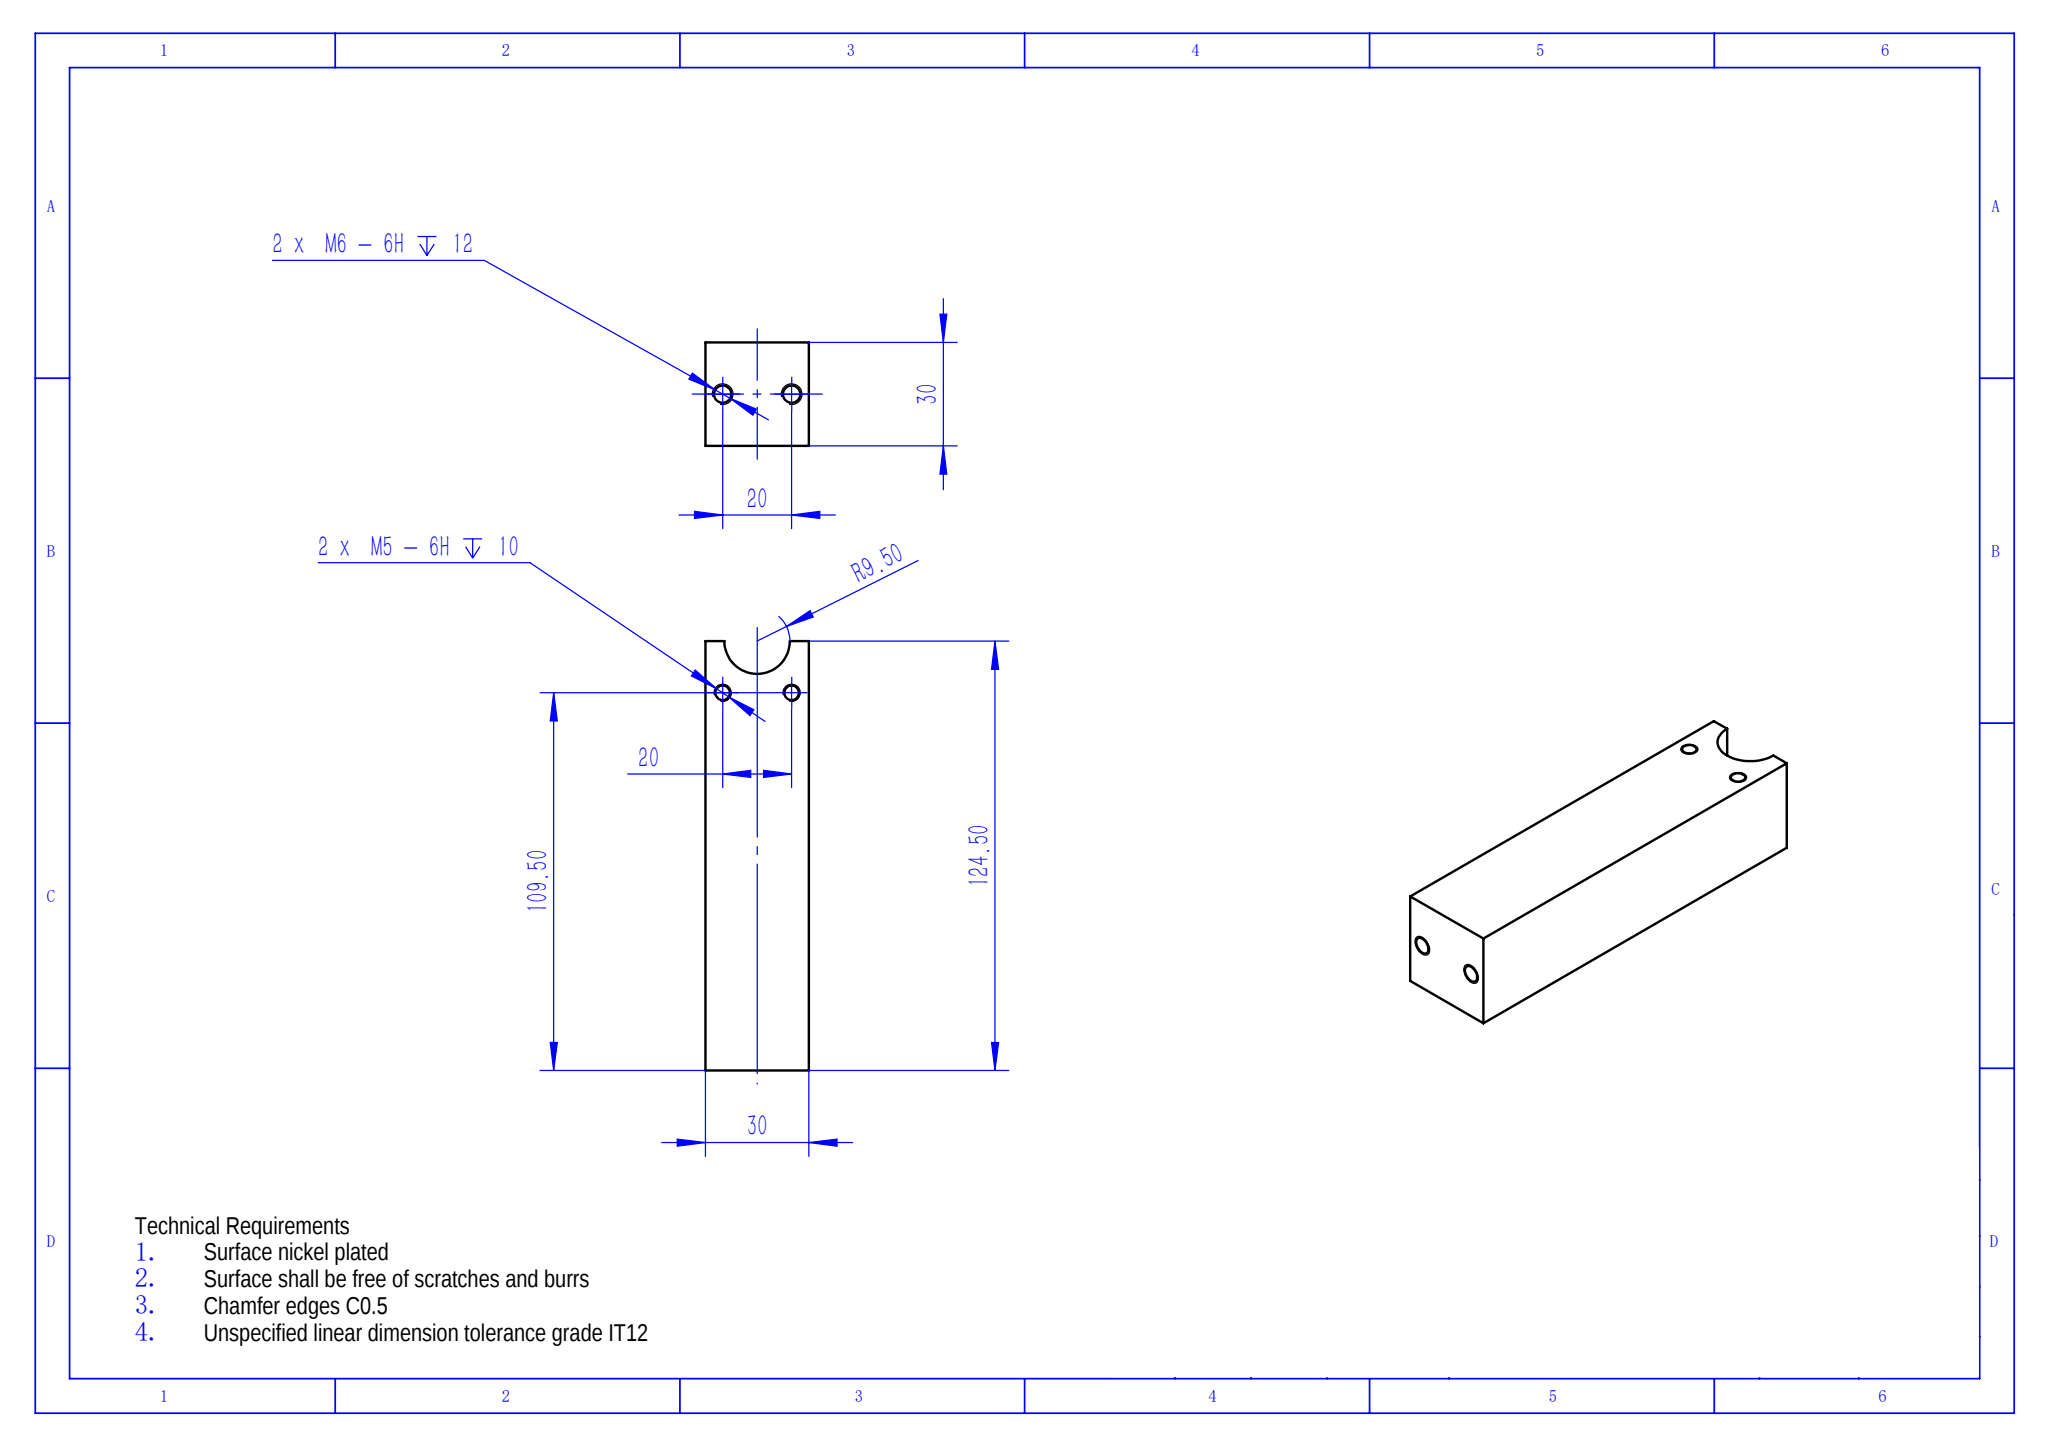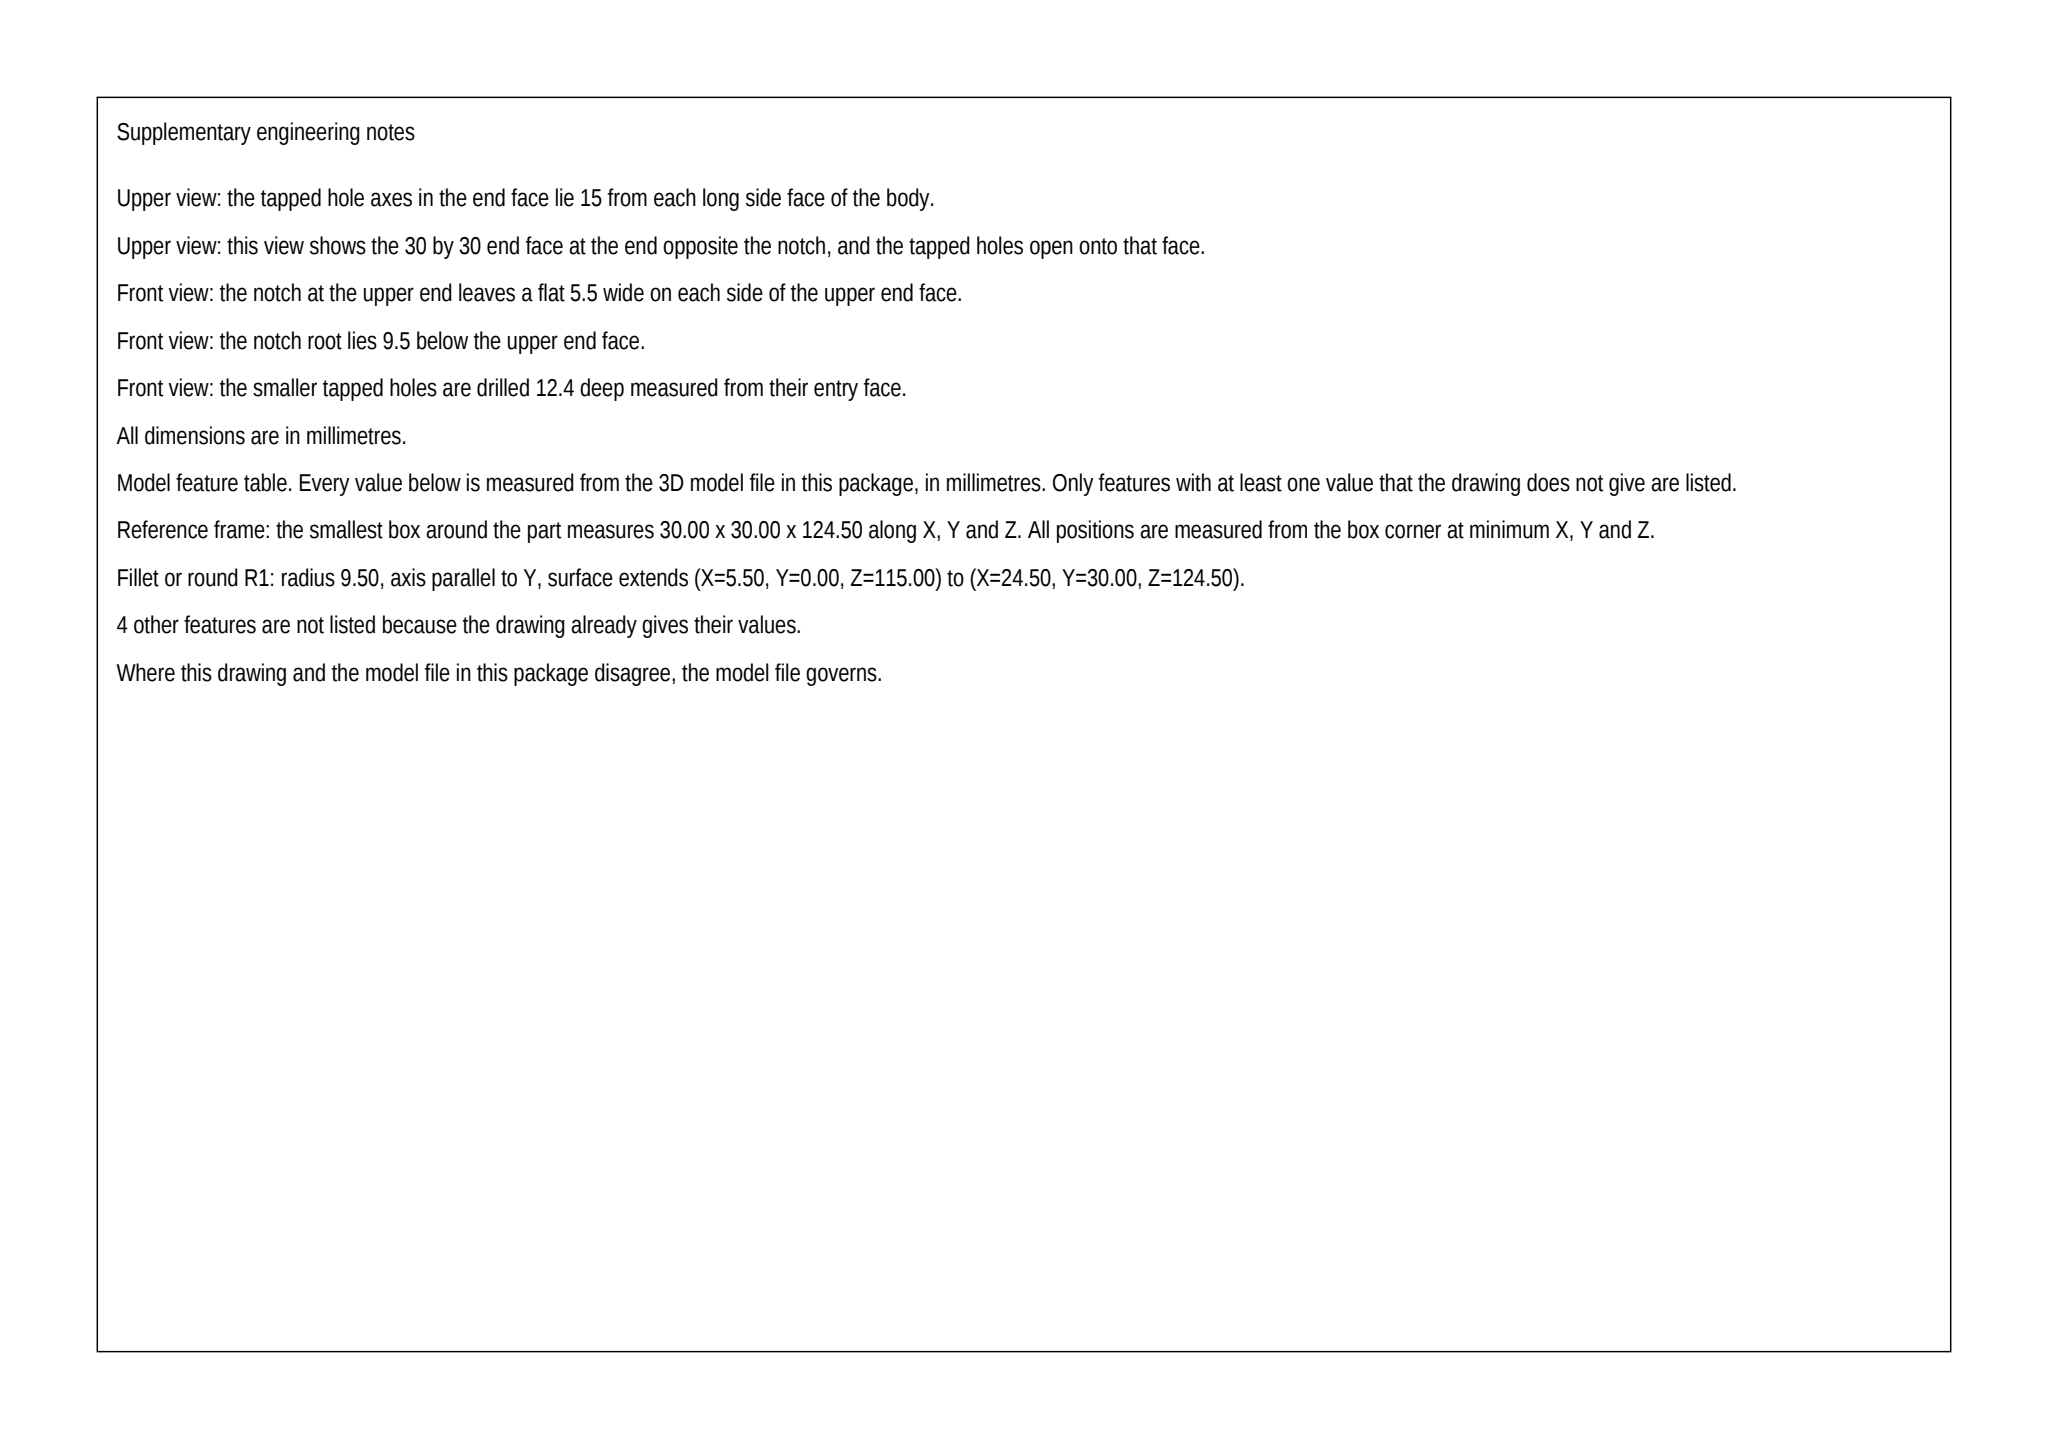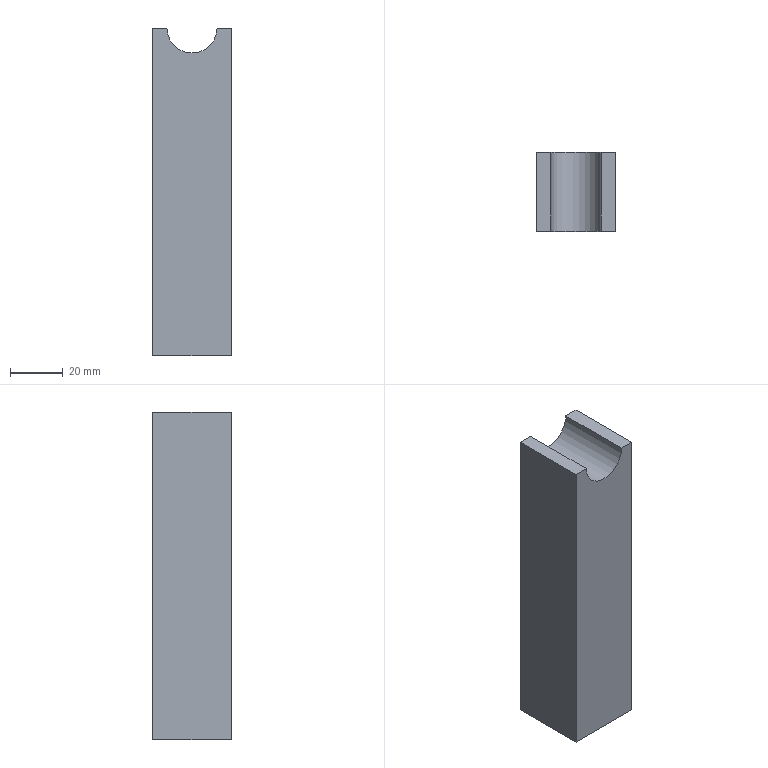Part | SolidWorks | mm | 1 solid | 24 faces | box 30 x 30 x 124.5 mm | volume 106833 mm3 | cylinder 9 | cone 8 | plane 7 | commonest cylinder face diameters 4.2 x4 5 x4 19 x1
build123d program:
from build123d import *

# Parameters (mm, degrees)
SKETCH1_W             = 30
SKETCH1_H             = 30
BOSS_EXTRUDE1_DEPTH   = 124.5
SKETCH2_R             = 9.5
CUT_EXTRUDE1_DEPTH    = 132.53
M6_TAPPED_HOLE1_D     = 5
M6_TAPPED_HOLE1_DEPTH = 15
M6_TAPPED_HOLE1_TIP   = 1.502
M5_TAPPED_HOLE1_D     = 4.2
M5_TAPPED_HOLE1_DEPTH = 12.4
M5_TAPPED_HOLE1_TIP   = 1.262


with BuildPart() as part:
    # Sketch1 → Boss-Extrude1 (new body)
    with BuildSketch(Plane.XY):
        with Locations((15, 15)):
            Rectangle(SKETCH1_W, SKETCH1_H)
    extrude(amount=BOSS_EXTRUDE1_DEPTH)

    # Sketch2 → Cut-Extrude1 (cut, through all)
    with BuildSketch(Plane(origin=(0, 30, 0), x_dir=(1, 0, 0), z_dir=(0, 1, 0))):
        with Locations((15, -124.5)):
            Circle(SKETCH2_R)
    extrude(amount=-CUT_EXTRUDE1_DEPTH, mode=Mode.SUBTRACT)

    # M6 Tapped Hole1
    with Locations(Plane(origin=(0, 0, 0), x_dir=(-1, 0, 0), z_dir=(0, 0, -1))):
        with Locations((-25, 15), (-5, 15)):
            Hole(M6_TAPPED_HOLE1_D / 2, depth=M6_TAPPED_HOLE1_DEPTH)
            with Locations((0, 0, -(M6_TAPPED_HOLE1_DEPTH + M6_TAPPED_HOLE1_TIP / 2))):  # 118° drill point
                Cone(0, M6_TAPPED_HOLE1_D / 2, M6_TAPPED_HOLE1_TIP, mode=Mode.SUBTRACT)

    # M5 Tapped Hole1
    with Locations(Plane(origin=(0, 30, 0), x_dir=(1, 0, 0), z_dir=(0, 1, 0))):
        with Locations((25, -109.5), (5, -109.5)):
            Hole(M5_TAPPED_HOLE1_D / 2, depth=M5_TAPPED_HOLE1_DEPTH)
            with Locations((0, 0, -(M5_TAPPED_HOLE1_DEPTH + M5_TAPPED_HOLE1_TIP / 2))):  # 118° drill point
                Cone(0, M5_TAPPED_HOLE1_D / 2, M5_TAPPED_HOLE1_TIP, mode=Mode.SUBTRACT)


solid = part.part
STEP:
#1=CARTESIAN_POINT('',(25.,17.6,107.4));
#2=VERTEX_POINT('',#1);
#3=CARTESIAN_POINT('',(25.,17.6,111.6));
#4=VERTEX_POINT('',#3);
#5=CARTESIAN_POINT('',(25.,17.6,109.5));
#6=DIRECTION('',(0.,1.,0.));
#7=DIRECTION('',(0.,0.,1.));
#8=AXIS2_PLACEMENT_3D('',#5,#6,#7);
#9=CIRCLE('',#8,2.1);
#10=EDGE_CURVE('',#2,#4,#9,.T.);
#11=ORIENTED_EDGE('',*,*,#10,.F.);
#12=CARTESIAN_POINT('',(25.,30.,107.4));
#13=VERTEX_POINT('',#12);
#14=CARTESIAN_POINT('',(25.,30.,107.4));
#15=DIRECTION('',(0.,1.,0.));
#16=VECTOR('',#15,1000.);
#17=LINE('',#14,#16);
#18=EDGE_CURVE('',#2,#13,#17,.T.);
#19=ORIENTED_EDGE('',*,*,#18,.T.);
#20=CARTESIAN_POINT('',(25.,30.,111.6));
#21=VERTEX_POINT('',#20);
#22=CARTESIAN_POINT('',(25.,30.,109.5));
#23=DIRECTION('',(0.,1.,0.));
#24=DIRECTION('',(0.,0.,1.));
#25=AXIS2_PLACEMENT_3D('',#22,#23,#24);
#26=CIRCLE('',#25,2.1);
#27=EDGE_CURVE('',#13,#21,#26,.T.);
#28=ORIENTED_EDGE('',*,*,#27,.T.);
#29=CARTESIAN_POINT('',(25.,30.,111.6));
#30=DIRECTION('',(0.,1.,0.));
#31=VECTOR('',#30,1000.);
#32=LINE('',#29,#31);
#33=EDGE_CURVE('',#4,#21,#32,.T.);
#34=ORIENTED_EDGE('',*,*,#33,.F.);
#35=EDGE_LOOP('',(#11,#19,#28,#34));
#36=FACE_OUTER_BOUND('',#35,.T.);
#37=CARTESIAN_POINT('',(25.,30.,109.5));
#38=DIRECTION('',(0.,1.,0.));
#39=DIRECTION('',(0.,0.,1.));
#40=AXIS2_PLACEMENT_3D('',#37,#38,#39);
#41=CYLINDRICAL_SURFACE('',#40,2.1);
#42=ADVANCED_FACE('',(#36),#41,.F.);
#43=CARTESIAN_POINT('',(25.,16.338,109.5));
#44=VERTEX_POINT('',#43);
#45=CARTESIAN_POINT('',(25.,17.6,111.6));
#46=DIRECTION('',(0.,0.515,0.8572));
#47=VECTOR('',#46,1000.);
#48=LINE('',#45,#47);
#49=EDGE_CURVE('',#44,#4,#48,.T.);
#50=ORIENTED_EDGE('',*,*,#49,.F.);
#51=CARTESIAN_POINT('',(25.,17.6,107.4));
#52=DIRECTION('',(0.,0.515,-0.8572));
#53=VECTOR('',#52,1000.);
#54=LINE('',#51,#53);
#55=EDGE_CURVE('',#44,#2,#54,.T.);
#56=ORIENTED_EDGE('',*,*,#55,.T.);
#57=ORIENTED_EDGE('',*,*,#10,.T.);
#58=EDGE_LOOP('',(#50,#56,#57));
#59=FACE_OUTER_BOUND('',#58,.T.);
#60=CARTESIAN_POINT('',(25.,17.6,109.5));
#61=DIRECTION('',(0.,1.,0.));
#62=DIRECTION('',(0.,0.,1.));
#63=AXIS2_PLACEMENT_3D('',#60,#61,#62);
#64=CONICAL_SURFACE('',#63,2.1,1.03);
#65=ADVANCED_FACE('',(#59),#64,.F.);
#66=CARTESIAN_POINT('',(5.,17.6,107.4));
#67=VERTEX_POINT('',#66);
#68=CARTESIAN_POINT('',(5.,17.6,111.6));
#69=VERTEX_POINT('',#68);
#70=CARTESIAN_POINT('',(5.,17.6,109.5));
#71=DIRECTION('',(0.,1.,0.));
#72=DIRECTION('',(0.,0.,1.));
#73=AXIS2_PLACEMENT_3D('',#70,#71,#72);
#74=CIRCLE('',#73,2.1);
#75=EDGE_CURVE('',#67,#69,#74,.T.);
#76=ORIENTED_EDGE('',*,*,#75,.F.);
#77=CARTESIAN_POINT('',(5.,30.,107.4));
#78=VERTEX_POINT('',#77);
#79=CARTESIAN_POINT('',(5.,30.,107.4));
#80=DIRECTION('',(0.,1.,0.));
#81=VECTOR('',#80,1000.);
#82=LINE('',#79,#81);
#83=EDGE_CURVE('',#67,#78,#82,.T.);
#84=ORIENTED_EDGE('',*,*,#83,.T.);
#85=CARTESIAN_POINT('',(5.,30.,111.6));
#86=VERTEX_POINT('',#85);
#87=CARTESIAN_POINT('',(5.,30.,109.5));
#88=DIRECTION('',(0.,1.,0.));
#89=DIRECTION('',(0.,0.,1.));
#90=AXIS2_PLACEMENT_3D('',#87,#88,#89);
#91=CIRCLE('',#90,2.1);
#92=EDGE_CURVE('',#78,#86,#91,.T.);
#93=ORIENTED_EDGE('',*,*,#92,.T.);
#94=CARTESIAN_POINT('',(5.,30.,111.6));
#95=DIRECTION('',(0.,1.,0.));
#96=VECTOR('',#95,1000.);
#97=LINE('',#94,#96);
#98=EDGE_CURVE('',#69,#86,#97,.T.);
#99=ORIENTED_EDGE('',*,*,#98,.F.);
#100=EDGE_LOOP('',(#76,#84,#93,#99));
#101=FACE_OUTER_BOUND('',#100,.T.);
#102=CARTESIAN_POINT('',(5.,30.,109.5));
#103=DIRECTION('',(0.,1.,0.));
#104=DIRECTION('',(0.,0.,1.));
#105=AXIS2_PLACEMENT_3D('',#102,#103,#104);
#106=CYLINDRICAL_SURFACE('',#105,2.1);
#107=ADVANCED_FACE('',(#101),#106,.F.);
#108=CARTESIAN_POINT('',(5.,16.338,109.5));
#109=VERTEX_POINT('',#108);
#110=CARTESIAN_POINT('',(5.,17.6,111.6));
#111=DIRECTION('',(0.,0.515,0.8572));
#112=VECTOR('',#111,1000.);
#113=LINE('',#110,#112);
#114=EDGE_CURVE('',#109,#69,#113,.T.);
#115=ORIENTED_EDGE('',*,*,#114,.F.);
#116=CARTESIAN_POINT('',(5.,17.6,107.4));
#117=DIRECTION('',(0.,0.515,-0.8572));
#118=VECTOR('',#117,1000.);
#119=LINE('',#116,#118);
#120=EDGE_CURVE('',#109,#67,#119,.T.);
#121=ORIENTED_EDGE('',*,*,#120,.T.);
#122=ORIENTED_EDGE('',*,*,#75,.T.);
#123=EDGE_LOOP('',(#115,#121,#122));
#124=FACE_OUTER_BOUND('',#123,.T.);
#125=CARTESIAN_POINT('',(5.,17.6,109.5));
#126=DIRECTION('',(0.,1.,0.));
#127=DIRECTION('',(0.,0.,1.));
#128=AXIS2_PLACEMENT_3D('',#125,#126,#127);
#129=CONICAL_SURFACE('',#128,2.1,1.03);
#130=ADVANCED_FACE('',(#124),#129,.F.);
#131=CARTESIAN_POINT('',(27.5,15.,15.));
#132=VERTEX_POINT('',#131);
#133=CARTESIAN_POINT('',(22.5,15.,15.));
#134=VERTEX_POINT('',#133);
#135=CARTESIAN_POINT('',(25.,15.,15.));
#136=DIRECTION('',(0.,0.,-1.));
#137=DIRECTION('',(-1.,0.,0.));
#138=AXIS2_PLACEMENT_3D('',#135,#136,#137);
#139=CIRCLE('',#138,2.5);
#140=EDGE_CURVE('',#132,#134,#139,.T.);
#141=ORIENTED_EDGE('',*,*,#140,.F.);
#142=CARTESIAN_POINT('',(27.5,15.,-0.));
#143=VERTEX_POINT('',#142);
#144=CARTESIAN_POINT('',(27.5,15.,0.));
#145=DIRECTION('',(0.,0.,-1.));
#146=VECTOR('',#145,1000.);
#147=LINE('',#144,#146);
#148=EDGE_CURVE('',#132,#143,#147,.T.);
#149=ORIENTED_EDGE('',*,*,#148,.T.);
#150=CARTESIAN_POINT('',(22.5,15.,-0.));
#151=VERTEX_POINT('',#150);
#152=CARTESIAN_POINT('',(25.,15.,-0.));
#153=DIRECTION('',(0.,0.,-1.));
#154=DIRECTION('',(-1.,0.,0.));
#155=AXIS2_PLACEMENT_3D('',#152,#153,#154);
#156=CIRCLE('',#155,2.5);
#157=EDGE_CURVE('',#143,#151,#156,.T.);
#158=ORIENTED_EDGE('',*,*,#157,.T.);
#159=CARTESIAN_POINT('',(22.5,15.,0.));
#160=DIRECTION('',(0.,0.,-1.));
#161=VECTOR('',#160,1000.);
#162=LINE('',#159,#161);
#163=EDGE_CURVE('',#134,#151,#162,.T.);
#164=ORIENTED_EDGE('',*,*,#163,.F.);
#165=EDGE_LOOP('',(#141,#149,#158,#164));
#166=FACE_OUTER_BOUND('',#165,.T.);
#167=CARTESIAN_POINT('',(25.,15.,0.));
#168=DIRECTION('',(0.,0.,-1.));
#169=DIRECTION('',(-1.,0.,0.));
#170=AXIS2_PLACEMENT_3D('',#167,#168,#169);
#171=CYLINDRICAL_SURFACE('',#170,2.5);
#172=ADVANCED_FACE('',(#166),#171,.F.);
#173=CARTESIAN_POINT('',(25.,15.,16.502));
#174=VERTEX_POINT('',#173);
#175=CARTESIAN_POINT('',(22.5,15.,15.));
#176=DIRECTION('',(-0.8572,0.,-0.515));
#177=VECTOR('',#176,1000.);
#178=LINE('',#175,#177);
#179=EDGE_CURVE('',#174,#134,#178,.T.);
#180=ORIENTED_EDGE('',*,*,#179,.F.);
#181=CARTESIAN_POINT('',(27.5,15.,15.));
#182=DIRECTION('',(0.8572,0.,-0.515));
#183=VECTOR('',#182,1000.);
#184=LINE('',#181,#183);
#185=EDGE_CURVE('',#174,#132,#184,.T.);
#186=ORIENTED_EDGE('',*,*,#185,.T.);
#187=ORIENTED_EDGE('',*,*,#140,.T.);
#188=EDGE_LOOP('',(#180,#186,#187));
#189=FACE_OUTER_BOUND('',#188,.T.);
#190=CARTESIAN_POINT('',(25.,15.,15.));
#191=DIRECTION('',(0.,0.,-1.));
#192=DIRECTION('',(-1.,0.,0.));
#193=AXIS2_PLACEMENT_3D('',#190,#191,#192);
#194=CONICAL_SURFACE('',#193,2.5,1.03);
#195=ADVANCED_FACE('',(#189),#194,.F.);
#196=CARTESIAN_POINT('',(7.5,15.,15.));
#197=VERTEX_POINT('',#196);
#198=CARTESIAN_POINT('',(2.5,15.,15.));
#199=VERTEX_POINT('',#198);
#200=CARTESIAN_POINT('',(5.,15.,15.));
#201=DIRECTION('',(0.,0.,-1.));
#202=DIRECTION('',(-1.,0.,0.));
#203=AXIS2_PLACEMENT_3D('',#200,#201,#202);
#204=CIRCLE('',#203,2.5);
#205=EDGE_CURVE('',#197,#199,#204,.T.);
#206=ORIENTED_EDGE('',*,*,#205,.F.);
#207=CARTESIAN_POINT('',(7.5,15.,-0.));
#208=VERTEX_POINT('',#207);
#209=CARTESIAN_POINT('',(7.5,15.,0.));
#210=DIRECTION('',(0.,0.,-1.));
#211=VECTOR('',#210,1000.);
#212=LINE('',#209,#211);
#213=EDGE_CURVE('',#197,#208,#212,.T.);
#214=ORIENTED_EDGE('',*,*,#213,.T.);
#215=CARTESIAN_POINT('',(2.5,15.,-0.));
#216=VERTEX_POINT('',#215);
#217=CARTESIAN_POINT('',(5.,15.,-0.));
#218=DIRECTION('',(0.,0.,-1.));
#219=DIRECTION('',(-1.,0.,0.));
#220=AXIS2_PLACEMENT_3D('',#217,#218,#219);
#221=CIRCLE('',#220,2.5);
#222=EDGE_CURVE('',#208,#216,#221,.T.);
#223=ORIENTED_EDGE('',*,*,#222,.T.);
#224=CARTESIAN_POINT('',(2.5,15.,0.));
#225=DIRECTION('',(0.,0.,-1.));
#226=VECTOR('',#225,1000.);
#227=LINE('',#224,#226);
#228=EDGE_CURVE('',#199,#216,#227,.T.);
#229=ORIENTED_EDGE('',*,*,#228,.F.);
#230=EDGE_LOOP('',(#206,#214,#223,#229));
#231=FACE_OUTER_BOUND('',#230,.T.);
#232=CARTESIAN_POINT('',(5.,15.,0.));
#233=DIRECTION('',(0.,0.,-1.));
#234=DIRECTION('',(-1.,0.,0.));
#235=AXIS2_PLACEMENT_3D('',#232,#233,#234);
#236=CYLINDRICAL_SURFACE('',#235,2.5);
#237=ADVANCED_FACE('',(#231),#236,.F.);
#238=CARTESIAN_POINT('',(5.,15.,16.502));
#239=VERTEX_POINT('',#238);
#240=CARTESIAN_POINT('',(2.5,15.,15.));
#241=DIRECTION('',(-0.8572,0.,-0.515));
#242=VECTOR('',#241,1000.);
#243=LINE('',#240,#242);
#244=EDGE_CURVE('',#239,#199,#243,.T.);
#245=ORIENTED_EDGE('',*,*,#244,.F.);
#246=CARTESIAN_POINT('',(7.5,15.,15.));
#247=DIRECTION('',(0.8572,0.,-0.515));
#248=VECTOR('',#247,1000.);
#249=LINE('',#246,#248);
#250=EDGE_CURVE('',#239,#197,#249,.T.);
#251=ORIENTED_EDGE('',*,*,#250,.T.);
#252=ORIENTED_EDGE('',*,*,#205,.T.);
#253=EDGE_LOOP('',(#245,#251,#252));
#254=FACE_OUTER_BOUND('',#253,.T.);
#255=CARTESIAN_POINT('',(5.,15.,15.));
#256=DIRECTION('',(0.,0.,-1.));
#257=DIRECTION('',(-1.,0.,0.));
#258=AXIS2_PLACEMENT_3D('',#255,#256,#257);
#259=CONICAL_SURFACE('',#258,2.5,1.03);
#260=ADVANCED_FACE('',(#254),#259,.F.);
#261=CARTESIAN_POINT('',(0.,0.,124.5));
#262=VERTEX_POINT('',#261);
#263=CARTESIAN_POINT('',(5.5,0.,124.5));
#264=VERTEX_POINT('',#263);
#265=CARTESIAN_POINT('',(0.,0.,124.5));
#266=DIRECTION('',(1.,0.,0.));
#267=VECTOR('',#266,1000.);
#268=LINE('',#265,#267);
#269=EDGE_CURVE('',#262,#264,#268,.T.);
#270=ORIENTED_EDGE('',*,*,#269,.T.);
#271=CARTESIAN_POINT('',(5.5,30.,124.5));
#272=VERTEX_POINT('',#271);
#273=CARTESIAN_POINT('',(5.5,0.,124.5));
#274=DIRECTION('',(0.,1.,0.));
#275=VECTOR('',#274,1000.);
#276=LINE('',#273,#275);
#277=EDGE_CURVE('',#264,#272,#276,.T.);
#278=ORIENTED_EDGE('',*,*,#277,.T.);
#279=CARTESIAN_POINT('',(0.,30.,124.5));
#280=VERTEX_POINT('',#279);
#281=CARTESIAN_POINT('',(0.,30.,124.5));
#282=DIRECTION('',(-1.,0.,0.));
#283=VECTOR('',#282,1000.);
#284=LINE('',#281,#283);
#285=EDGE_CURVE('',#272,#280,#284,.T.);
#286=ORIENTED_EDGE('',*,*,#285,.T.);
#287=CARTESIAN_POINT('',(0.,0.,124.5));
#288=DIRECTION('',(0.,-1.,0.));
#289=VECTOR('',#288,1000.);
#290=LINE('',#287,#289);
#291=EDGE_CURVE('',#280,#262,#290,.T.);
#292=ORIENTED_EDGE('',*,*,#291,.T.);
#293=EDGE_LOOP('',(#270,#278,#286,#292));
#294=FACE_OUTER_BOUND('',#293,.T.);
#295=CARTESIAN_POINT('',(0.,0.,124.5));
#296=DIRECTION('',(0.,0.,-1.));
#297=DIRECTION('',(-1.,0.,0.));
#298=AXIS2_PLACEMENT_3D('',#295,#296,#297);
#299=PLANE('',#298);
#300=ADVANCED_FACE('',(#294),#299,.F.);
#301=CARTESIAN_POINT('',(0.,30.,0.));
#302=VERTEX_POINT('',#301);
#303=CARTESIAN_POINT('',(0.,0.,0.));
#304=VERTEX_POINT('',#303);
#305=CARTESIAN_POINT('',(0.,0.,0.));
#306=DIRECTION('',(0.,-1.,0.));
#307=VECTOR('',#306,1000.);
#308=LINE('',#305,#307);
#309=EDGE_CURVE('',#302,#304,#308,.T.);
#310=ORIENTED_EDGE('',*,*,#309,.T.);
#311=CARTESIAN_POINT('',(0.,0.,124.5));
#312=DIRECTION('',(0.,0.,-1.));
#313=VECTOR('',#312,1000.);
#314=LINE('',#311,#313);
#315=EDGE_CURVE('',#262,#304,#314,.T.);
#316=ORIENTED_EDGE('',*,*,#315,.F.);
#317=ORIENTED_EDGE('',*,*,#291,.F.);
#318=CARTESIAN_POINT('',(0.,30.,124.5));
#319=DIRECTION('',(0.,0.,-1.));
#320=VECTOR('',#319,1000.);
#321=LINE('',#318,#320);
#322=EDGE_CURVE('',#280,#302,#321,.T.);
#323=ORIENTED_EDGE('',*,*,#322,.T.);
#324=EDGE_LOOP('',(#310,#316,#317,#323));
#325=FACE_OUTER_BOUND('',#324,.T.);
#326=CARTESIAN_POINT('',(0.,0.,124.5));
#327=DIRECTION('',(1.,0.,0.));
#328=DIRECTION('',(0.,0.,-1.));
#329=AXIS2_PLACEMENT_3D('',#326,#327,#328);
#330=PLANE('',#329);
#331=ADVANCED_FACE('',(#325),#330,.F.);
#332=CARTESIAN_POINT('',(24.5,0.,124.5));
#333=VERTEX_POINT('',#332);
#334=CARTESIAN_POINT('',(30.,0.,124.5));
#335=VERTEX_POINT('',#334);
#336=CARTESIAN_POINT('',(0.,0.,124.5));
#337=DIRECTION('',(1.,0.,0.));
#338=VECTOR('',#337,1000.);
#339=LINE('',#336,#338);
#340=EDGE_CURVE('',#333,#335,#339,.T.);
#341=ORIENTED_EDGE('',*,*,#340,.F.);
#342=CARTESIAN_POINT('',(15.,0.,124.5));
#343=DIRECTION('',(0.,1.,0.));
#344=DIRECTION('',(0.,0.,1.));
#345=AXIS2_PLACEMENT_3D('',#342,#343,#344);
#346=CIRCLE('',#345,9.5);
#347=EDGE_CURVE('',#333,#264,#346,.T.);
#348=ORIENTED_EDGE('',*,*,#347,.T.);
#349=ORIENTED_EDGE('',*,*,#269,.F.);
#350=ORIENTED_EDGE('',*,*,#315,.T.);
#351=CARTESIAN_POINT('',(30.,0.,0.));
#352=VERTEX_POINT('',#351);
#353=CARTESIAN_POINT('',(0.,0.,0.));
#354=DIRECTION('',(1.,0.,0.));
#355=VECTOR('',#354,1000.);
#356=LINE('',#353,#355);
#357=EDGE_CURVE('',#304,#352,#356,.T.);
#358=ORIENTED_EDGE('',*,*,#357,.T.);
#359=CARTESIAN_POINT('',(30.,0.,124.5));
#360=DIRECTION('',(0.,0.,-1.));
#361=VECTOR('',#360,1000.);
#362=LINE('',#359,#361);
#363=EDGE_CURVE('',#335,#352,#362,.T.);
#364=ORIENTED_EDGE('',*,*,#363,.F.);
#365=EDGE_LOOP('',(#341,#348,#349,#350,#358,#364));
#366=FACE_OUTER_BOUND('',#365,.T.);
#367=CARTESIAN_POINT('',(0.,0.,124.5));
#368=DIRECTION('',(0.,1.,0.));
#369=DIRECTION('',(0.,0.,1.));
#370=AXIS2_PLACEMENT_3D('',#367,#368,#369);
#371=PLANE('',#370);
#372=ADVANCED_FACE('',(#366),#371,.F.);
#373=CARTESIAN_POINT('',(30.,30.,0.));
#374=VERTEX_POINT('',#373);
#375=CARTESIAN_POINT('',(30.,0.,0.));
#376=DIRECTION('',(0.,1.,0.));
#377=VECTOR('',#376,1000.);
#378=LINE('',#375,#377);
#379=EDGE_CURVE('',#352,#374,#378,.T.);
#380=ORIENTED_EDGE('',*,*,#379,.T.);
#381=CARTESIAN_POINT('',(30.,30.,124.5));
#382=VERTEX_POINT('',#381);
#383=CARTESIAN_POINT('',(30.,30.,124.5));
#384=DIRECTION('',(0.,0.,-1.));
#385=VECTOR('',#384,1000.);
#386=LINE('',#383,#385);
#387=EDGE_CURVE('',#382,#374,#386,.T.);
#388=ORIENTED_EDGE('',*,*,#387,.F.);
#389=CARTESIAN_POINT('',(30.,0.,124.5));
#390=DIRECTION('',(0.,1.,0.));
#391=VECTOR('',#390,1000.);
#392=LINE('',#389,#391);
#393=EDGE_CURVE('',#335,#382,#392,.T.);
#394=ORIENTED_EDGE('',*,*,#393,.F.);
#395=ORIENTED_EDGE('',*,*,#363,.T.);
#396=EDGE_LOOP('',(#380,#388,#394,#395));
#397=FACE_OUTER_BOUND('',#396,.T.);
#398=CARTESIAN_POINT('',(30.,0.,124.5));
#399=DIRECTION('',(-1.,0.,0.));
#400=DIRECTION('',(0.,0.,1.));
#401=AXIS2_PLACEMENT_3D('',#398,#399,#400);
#402=PLANE('',#401);
#403=ADVANCED_FACE('',(#397),#402,.F.);
#404=CARTESIAN_POINT('',(25.,30.,109.5));
#405=DIRECTION('',(0.,1.,0.));
#406=DIRECTION('',(0.,0.,1.));
#407=AXIS2_PLACEMENT_3D('',#404,#405,#406);
#408=CIRCLE('',#407,2.1);
#409=EDGE_CURVE('',#21,#13,#408,.T.);
#410=ORIENTED_EDGE('',*,*,#409,.F.);
#411=ORIENTED_EDGE('',*,*,#27,.F.);
#412=EDGE_LOOP('',(#410,#411));
#413=FACE_BOUND('',#412,.T.);
#414=CARTESIAN_POINT('',(5.,30.,109.5));
#415=DIRECTION('',(0.,1.,0.));
#416=DIRECTION('',(0.,0.,1.));
#417=AXIS2_PLACEMENT_3D('',#414,#415,#416);
#418=CIRCLE('',#417,2.1);
#419=EDGE_CURVE('',#86,#78,#418,.T.);
#420=ORIENTED_EDGE('',*,*,#419,.F.);
#421=ORIENTED_EDGE('',*,*,#92,.F.);
#422=EDGE_LOOP('',(#420,#421));
#423=FACE_BOUND('',#422,.T.);
#424=ORIENTED_EDGE('',*,*,#285,.F.);
#425=CARTESIAN_POINT('',(24.5,30.,124.5));
#426=VERTEX_POINT('',#425);
#427=CARTESIAN_POINT('',(15.,30.,124.5));
#428=DIRECTION('',(0.,1.,0.));
#429=DIRECTION('',(0.,0.,1.));
#430=AXIS2_PLACEMENT_3D('',#427,#428,#429);
#431=CIRCLE('',#430,9.5);
#432=EDGE_CURVE('',#426,#272,#431,.T.);
#433=ORIENTED_EDGE('',*,*,#432,.F.);
#434=CARTESIAN_POINT('',(0.,30.,124.5));
#435=DIRECTION('',(-1.,0.,0.));
#436=VECTOR('',#435,1000.);
#437=LINE('',#434,#436);
#438=EDGE_CURVE('',#382,#426,#437,.T.);
#439=ORIENTED_EDGE('',*,*,#438,.F.);
#440=ORIENTED_EDGE('',*,*,#387,.T.);
#441=CARTESIAN_POINT('',(0.,30.,0.));
#442=DIRECTION('',(-1.,0.,0.));
#443=VECTOR('',#442,1000.);
#444=LINE('',#441,#443);
#445=EDGE_CURVE('',#374,#302,#444,.T.);
#446=ORIENTED_EDGE('',*,*,#445,.T.);
#447=ORIENTED_EDGE('',*,*,#322,.F.);
#448=EDGE_LOOP('',(#424,#433,#439,#440,#446,#447));
#449=FACE_OUTER_BOUND('',#448,.T.);
#450=CARTESIAN_POINT('',(0.,30.,124.5));
#451=DIRECTION('',(0.,-1.,0.));
#452=DIRECTION('',(0.,0.,-1.));
#453=AXIS2_PLACEMENT_3D('',#450,#451,#452);
#454=PLANE('',#453);
#455=ADVANCED_FACE('',(#413,#423,#449),#454,.F.);
#456=ORIENTED_EDGE('',*,*,#438,.T.);
#457=CARTESIAN_POINT('',(24.5,0.,124.5));
#458=DIRECTION('',(0.,-1.,0.));
#459=VECTOR('',#458,1000.);
#460=LINE('',#457,#459);
#461=EDGE_CURVE('',#426,#333,#460,.T.);
#462=ORIENTED_EDGE('',*,*,#461,.T.);
#463=ORIENTED_EDGE('',*,*,#340,.T.);
#464=ORIENTED_EDGE('',*,*,#393,.T.);
#465=EDGE_LOOP('',(#456,#462,#463,#464));
#466=FACE_OUTER_BOUND('',#465,.T.);
#467=CARTESIAN_POINT('',(0.,0.,124.5));
#468=DIRECTION('',(0.,0.,-1.));
#469=DIRECTION('',(-1.,0.,0.));
#470=AXIS2_PLACEMENT_3D('',#467,#468,#469);
#471=PLANE('',#470);
#472=ADVANCED_FACE('',(#466),#471,.F.);
#473=CARTESIAN_POINT('',(25.,15.,-0.));
#474=DIRECTION('',(0.,0.,-1.));
#475=DIRECTION('',(-1.,0.,0.));
#476=AXIS2_PLACEMENT_3D('',#473,#474,#475);
#477=CIRCLE('',#476,2.5);
#478=EDGE_CURVE('',#151,#143,#477,.T.);
#479=ORIENTED_EDGE('',*,*,#478,.F.);
#480=ORIENTED_EDGE('',*,*,#157,.F.);
#481=EDGE_LOOP('',(#479,#480));
#482=FACE_BOUND('',#481,.T.);
#483=CARTESIAN_POINT('',(5.,15.,-0.));
#484=DIRECTION('',(0.,0.,-1.));
#485=DIRECTION('',(-1.,0.,0.));
#486=AXIS2_PLACEMENT_3D('',#483,#484,#485);
#487=CIRCLE('',#486,2.5);
#488=EDGE_CURVE('',#216,#208,#487,.T.);
#489=ORIENTED_EDGE('',*,*,#488,.F.);
#490=ORIENTED_EDGE('',*,*,#222,.F.);
#491=EDGE_LOOP('',(#489,#490));
#492=FACE_BOUND('',#491,.T.);
#493=ORIENTED_EDGE('',*,*,#309,.F.);
#494=ORIENTED_EDGE('',*,*,#445,.F.);
#495=ORIENTED_EDGE('',*,*,#379,.F.);
#496=ORIENTED_EDGE('',*,*,#357,.F.);
#497=EDGE_LOOP('',(#493,#494,#495,#496));
#498=FACE_OUTER_BOUND('',#497,.T.);
#499=CARTESIAN_POINT('',(0.,0.,0.));
#500=DIRECTION('',(0.,0.,-1.));
#501=DIRECTION('',(-1.,0.,0.));
#502=AXIS2_PLACEMENT_3D('',#499,#500,#501);
#503=PLANE('',#502);
#504=ADVANCED_FACE('',(#482,#492,#498),#503,.T.);
#505=ORIENTED_EDGE('',*,*,#347,.F.);
#506=ORIENTED_EDGE('',*,*,#461,.F.);
#507=ORIENTED_EDGE('',*,*,#432,.T.);
#508=ORIENTED_EDGE('',*,*,#277,.F.);
#509=EDGE_LOOP('',(#505,#506,#507,#508));
#510=FACE_OUTER_BOUND('',#509,.T.);
#511=CARTESIAN_POINT('',(15.,0.,124.5));
#512=DIRECTION('',(0.,1.,0.));
#513=DIRECTION('',(0.,0.,1.));
#514=AXIS2_PLACEMENT_3D('',#511,#512,#513);
#515=CYLINDRICAL_SURFACE('',#514,9.5);
#516=ADVANCED_FACE('',(#510),#515,.F.);
#517=ORIENTED_EDGE('',*,*,#250,.F.);
#518=ORIENTED_EDGE('',*,*,#244,.T.);
#519=CARTESIAN_POINT('',(5.,15.,15.));
#520=DIRECTION('',(0.,0.,-1.));
#521=DIRECTION('',(-1.,0.,0.));
#522=AXIS2_PLACEMENT_3D('',#519,#520,#521);
#523=CIRCLE('',#522,2.5);
#524=EDGE_CURVE('',#199,#197,#523,.T.);
#525=ORIENTED_EDGE('',*,*,#524,.T.);
#526=EDGE_LOOP('',(#517,#518,#525));
#527=FACE_OUTER_BOUND('',#526,.T.);
#528=CARTESIAN_POINT('',(5.,15.,15.));
#529=DIRECTION('',(0.,0.,-1.));
#530=DIRECTION('',(-1.,0.,0.));
#531=AXIS2_PLACEMENT_3D('',#528,#529,#530);
#532=CONICAL_SURFACE('',#531,2.5,1.03);
#533=ADVANCED_FACE('',(#527),#532,.F.);
#534=ORIENTED_EDGE('',*,*,#213,.F.);
#535=ORIENTED_EDGE('',*,*,#524,.F.);
#536=ORIENTED_EDGE('',*,*,#228,.T.);
#537=ORIENTED_EDGE('',*,*,#488,.T.);
#538=EDGE_LOOP('',(#534,#535,#536,#537));
#539=FACE_OUTER_BOUND('',#538,.T.);
#540=CARTESIAN_POINT('',(5.,15.,0.));
#541=DIRECTION('',(0.,0.,-1.));
#542=DIRECTION('',(-1.,0.,0.));
#543=AXIS2_PLACEMENT_3D('',#540,#541,#542);
#544=CYLINDRICAL_SURFACE('',#543,2.5);
#545=ADVANCED_FACE('',(#539),#544,.F.);
#546=ORIENTED_EDGE('',*,*,#185,.F.);
#547=ORIENTED_EDGE('',*,*,#179,.T.);
#548=CARTESIAN_POINT('',(25.,15.,15.));
#549=DIRECTION('',(0.,0.,-1.));
#550=DIRECTION('',(-1.,0.,0.));
#551=AXIS2_PLACEMENT_3D('',#548,#549,#550);
#552=CIRCLE('',#551,2.5);
#553=EDGE_CURVE('',#134,#132,#552,.T.);
#554=ORIENTED_EDGE('',*,*,#553,.T.);
#555=EDGE_LOOP('',(#546,#547,#554));
#556=FACE_OUTER_BOUND('',#555,.T.);
#557=CARTESIAN_POINT('',(25.,15.,15.));
#558=DIRECTION('',(0.,0.,-1.));
#559=DIRECTION('',(-1.,0.,0.));
#560=AXIS2_PLACEMENT_3D('',#557,#558,#559);
#561=CONICAL_SURFACE('',#560,2.5,1.03);
#562=ADVANCED_FACE('',(#556),#561,.F.);
#563=ORIENTED_EDGE('',*,*,#148,.F.);
#564=ORIENTED_EDGE('',*,*,#553,.F.);
#565=ORIENTED_EDGE('',*,*,#163,.T.);
#566=ORIENTED_EDGE('',*,*,#478,.T.);
#567=EDGE_LOOP('',(#563,#564,#565,#566));
#568=FACE_OUTER_BOUND('',#567,.T.);
#569=CARTESIAN_POINT('',(25.,15.,0.));
#570=DIRECTION('',(0.,0.,-1.));
#571=DIRECTION('',(-1.,0.,0.));
#572=AXIS2_PLACEMENT_3D('',#569,#570,#571);
#573=CYLINDRICAL_SURFACE('',#572,2.5);
#574=ADVANCED_FACE('',(#568),#573,.F.);
#575=ORIENTED_EDGE('',*,*,#120,.F.);
#576=ORIENTED_EDGE('',*,*,#114,.T.);
#577=CARTESIAN_POINT('',(5.,17.6,109.5));
#578=DIRECTION('',(0.,1.,0.));
#579=DIRECTION('',(0.,0.,1.));
#580=AXIS2_PLACEMENT_3D('',#577,#578,#579);
#581=CIRCLE('',#580,2.1);
#582=EDGE_CURVE('',#69,#67,#581,.T.);
#583=ORIENTED_EDGE('',*,*,#582,.T.);
#584=EDGE_LOOP('',(#575,#576,#583));
#585=FACE_OUTER_BOUND('',#584,.T.);
#586=CARTESIAN_POINT('',(5.,17.6,109.5));
#587=DIRECTION('',(0.,1.,0.));
#588=DIRECTION('',(0.,0.,1.));
#589=AXIS2_PLACEMENT_3D('',#586,#587,#588);
#590=CONICAL_SURFACE('',#589,2.1,1.03);
#591=ADVANCED_FACE('',(#585),#590,.F.);
#592=ORIENTED_EDGE('',*,*,#83,.F.);
#593=ORIENTED_EDGE('',*,*,#582,.F.);
#594=ORIENTED_EDGE('',*,*,#98,.T.);
#595=ORIENTED_EDGE('',*,*,#419,.T.);
#596=EDGE_LOOP('',(#592,#593,#594,#595));
#597=FACE_OUTER_BOUND('',#596,.T.);
#598=CARTESIAN_POINT('',(5.,30.,109.5));
#599=DIRECTION('',(0.,1.,0.));
#600=DIRECTION('',(0.,0.,1.));
#601=AXIS2_PLACEMENT_3D('',#598,#599,#600);
#602=CYLINDRICAL_SURFACE('',#601,2.1);
#603=ADVANCED_FACE('',(#597),#602,.F.);
#604=ORIENTED_EDGE('',*,*,#55,.F.);
#605=ORIENTED_EDGE('',*,*,#49,.T.);
#606=CARTESIAN_POINT('',(25.,17.6,109.5));
#607=DIRECTION('',(0.,1.,0.));
#608=DIRECTION('',(0.,0.,1.));
#609=AXIS2_PLACEMENT_3D('',#606,#607,#608);
#610=CIRCLE('',#609,2.1);
#611=EDGE_CURVE('',#4,#2,#610,.T.);
#612=ORIENTED_EDGE('',*,*,#611,.T.);
#613=EDGE_LOOP('',(#604,#605,#612));
#614=FACE_OUTER_BOUND('',#613,.T.);
#615=CARTESIAN_POINT('',(25.,17.6,109.5));
#616=DIRECTION('',(0.,1.,0.));
#617=DIRECTION('',(0.,0.,1.));
#618=AXIS2_PLACEMENT_3D('',#615,#616,#617);
#619=CONICAL_SURFACE('',#618,2.1,1.03);
#620=ADVANCED_FACE('',(#614),#619,.F.);
#621=ORIENTED_EDGE('',*,*,#18,.F.);
#622=ORIENTED_EDGE('',*,*,#611,.F.);
#623=ORIENTED_EDGE('',*,*,#33,.T.);
#624=ORIENTED_EDGE('',*,*,#409,.T.);
#625=EDGE_LOOP('',(#621,#622,#623,#624));
#626=FACE_OUTER_BOUND('',#625,.T.);
#627=CARTESIAN_POINT('',(25.,30.,109.5));
#628=DIRECTION('',(0.,1.,0.));
#629=DIRECTION('',(0.,0.,1.));
#630=AXIS2_PLACEMENT_3D('',#627,#628,#629);
#631=CYLINDRICAL_SURFACE('',#630,2.1);
#632=ADVANCED_FACE('',(#626),#631,.F.);
#633=CLOSED_SHELL('',(#42,#65,#107,#130,#172,#195,#237,#260,#300,#331,#372,#403,#455,#472,#504,#516,#533,#545,#562,#574,#591,#603,#620,#632));
#634=MANIFOLD_SOLID_BREP('',#633);
#635=CARTESIAN_POINT('',(0.,0.,0.));
#636=DIRECTION('',(0.,0.,1.));
#637=DIRECTION('',(1.,0.,0.));
#638=AXIS2_PLACEMENT_3D('',#635,#636,#637);
#639=(LENGTH_UNIT()NAMED_UNIT(*)SI_UNIT(.MILLI.,.METRE.));
#640=UNCERTAINTY_MEASURE_WITH_UNIT(LENGTH_MEASURE(0.00001),#639,'','');
#641=(NAMED_UNIT(*)PLANE_ANGLE_UNIT()SI_UNIT($,.RADIAN.));
#642=(NAMED_UNIT(*)SI_UNIT($,.STERADIAN.)SOLID_ANGLE_UNIT());
#643=(GEOMETRIC_REPRESENTATION_CONTEXT(3)GLOBAL_UNCERTAINTY_ASSIGNED_CONTEXT((#640))GLOBAL_UNIT_ASSIGNED_CONTEXT((#639,#641,#642))REPRESENTATION_CONTEXT('',''));
#644=ADVANCED_BREP_SHAPE_REPRESENTATION('',(#634,#638),#643);